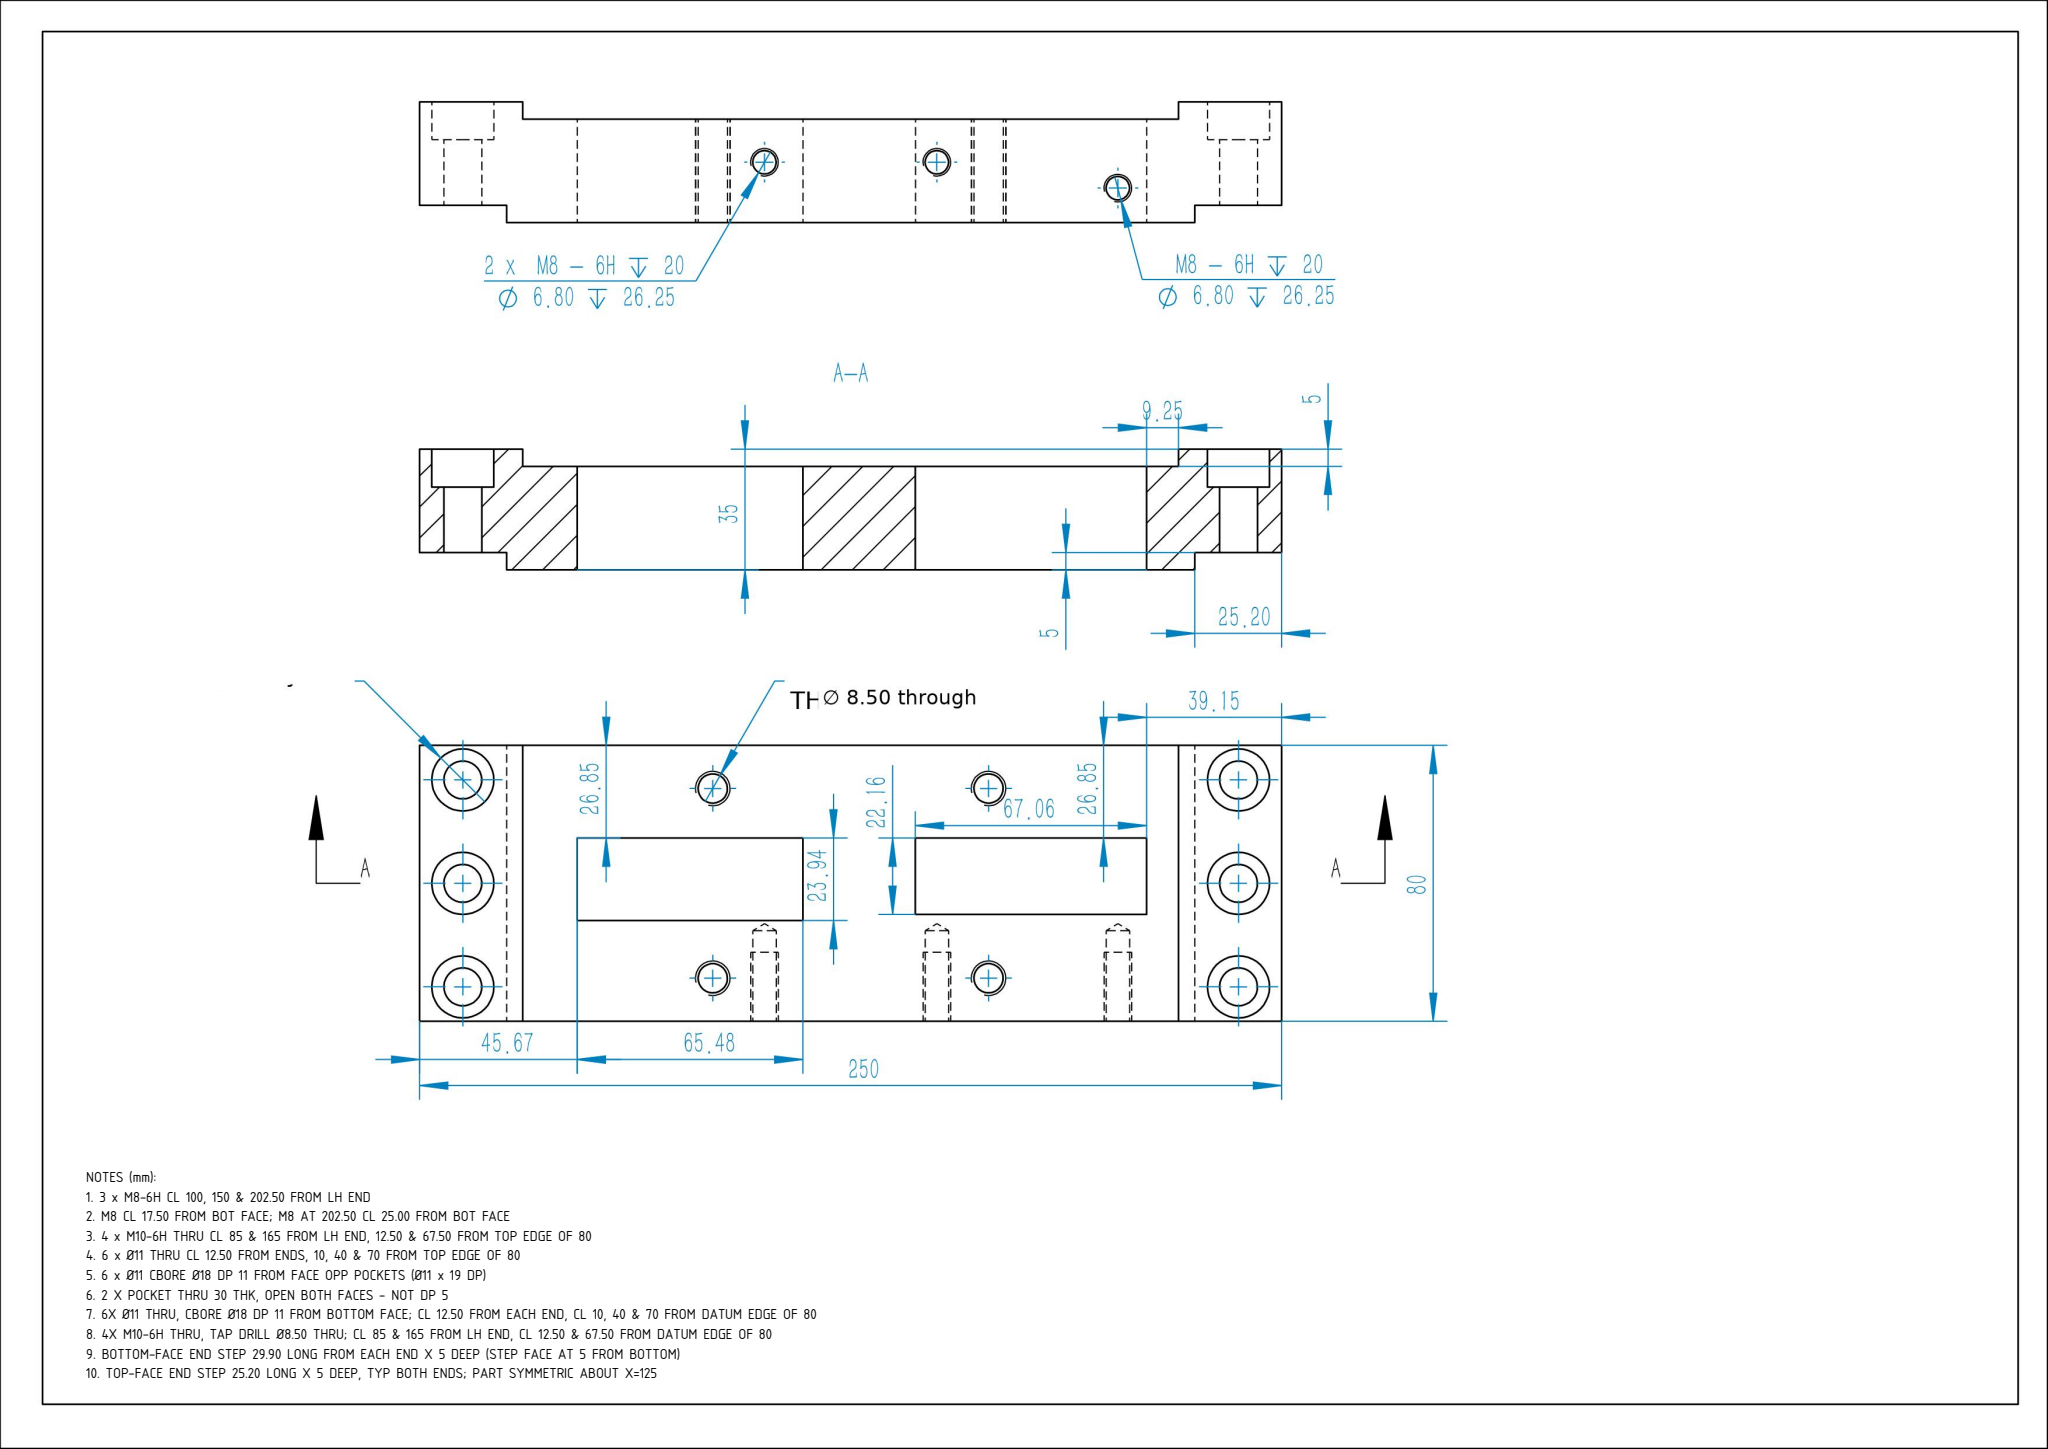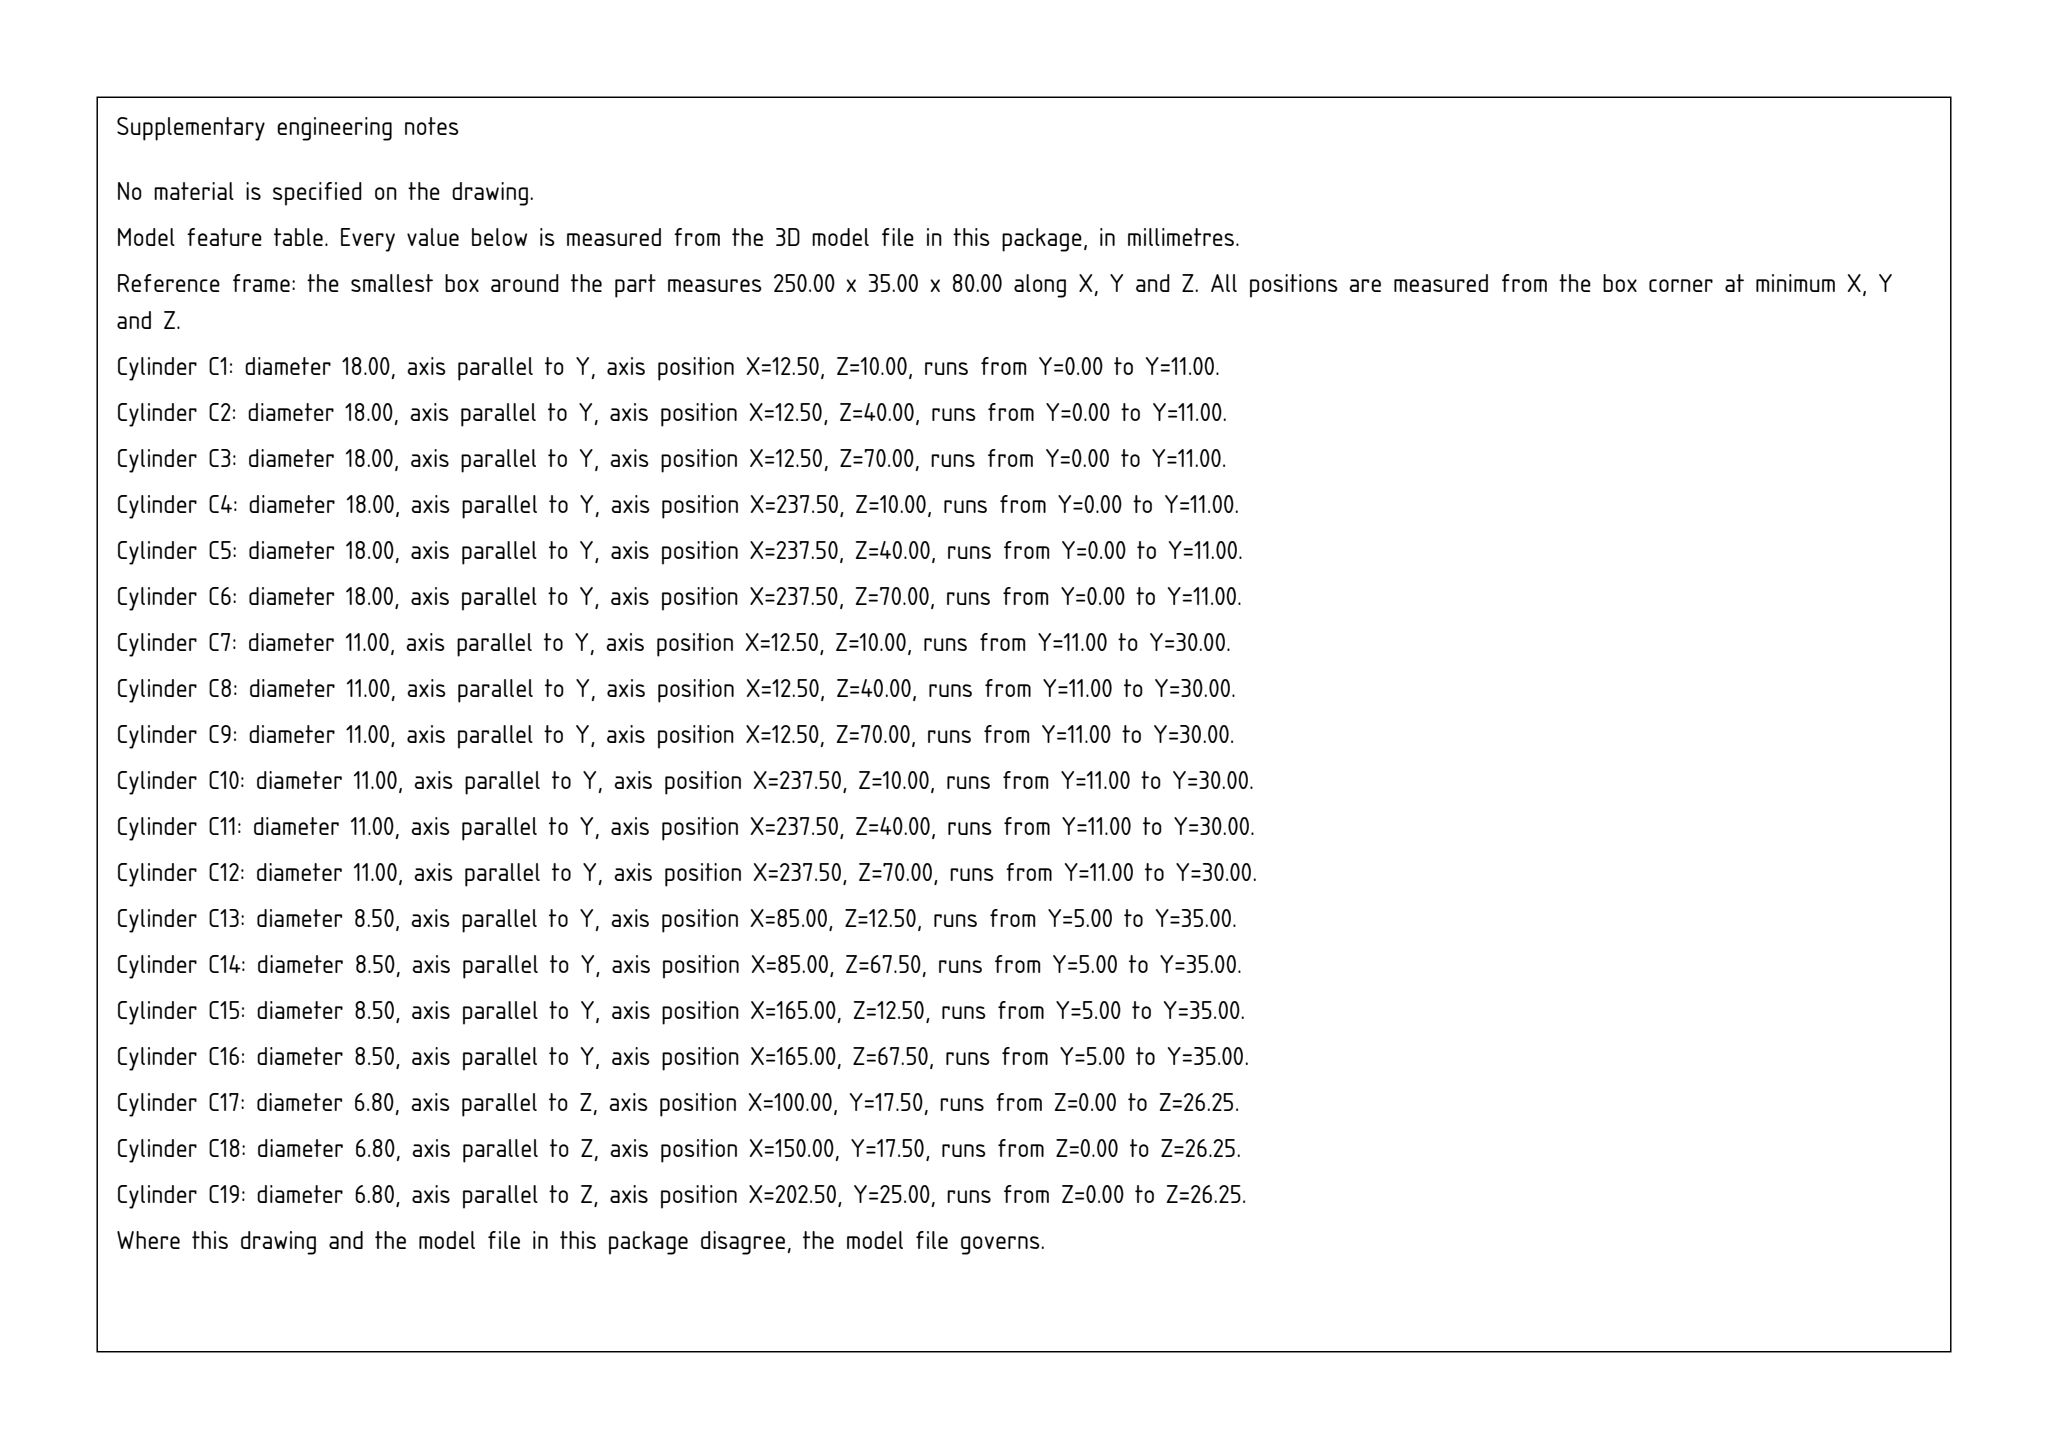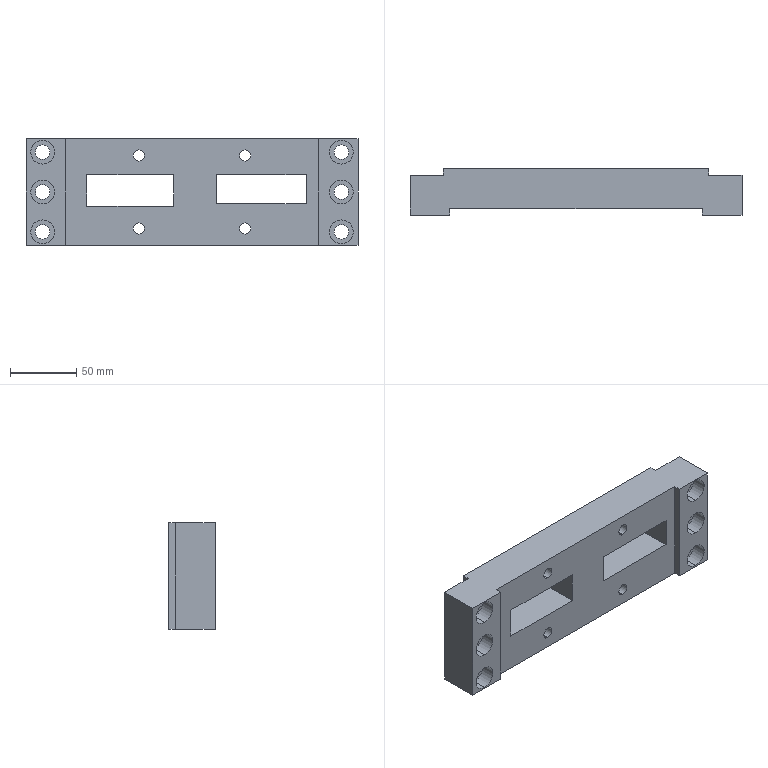Part | SolidWorks | mm | 1 solid | 72 faces | box 250 x 35 x 80 mm | volume 474796 mm3 | cylinder 38 | plane 28 | cone 6 | commonest cylinder face diameters 18 x12 11 x12 8.5 x8 6.8 x6
Drawing notes:
3 x M8-6H CL 100, 150 & 202.50 FROM LH END | from the solid: Ø6.80 cyls axis z at x=100, 150, 202.5, len 26.25
M8 CL 17.50 FROM BOT FACE; M8 AT 202.50 CL 25.00 FROM BOT FACE | from the solid: Ø6.80 axis z at y=17.5 (x100,150) and y=25.0 (x202.5)
4 x M10-6H THRU CL 85 & 165 FROM LH END, 12.50 & 67.50 FROM TOP EDGE OF 80 | from the solid: Ø8.5 axis y cyls at (85,12.5),(85,67.5),(165,12.5),(165,67.5), len 30
6 x Ø11 THRU CL 12.50 FROM ENDS, 10, 40 & 70 FROM TOP EDGE OF 80 | from the solid: Ø11 axis y cyls at x=12.5 & 237.5, z=10/40/70
6 x Ø11 CBORE Ø18 DP 11 FROM FACE OPP POCKETS (Ø11 x 19 DP) | from the solid: Ø18 cyl len 11 coaxial with Ø11 len 19; y-planes 0 & 11 (6 faces)
2 X POCKET THRU 30 THK, OPEN BOTH FACES - NOT DP 5 | from the solid: Pocket walls x45.7-111.2 & x143.8-210.9 span y 5.0 to 35.0 (full 30 web); floors only at z29.2/31.0 & 53.2, no y-floor face
6X Ø11 THRU, CBORE Ø18 DP 11 FROM BOTTOM FACE; CL 12.50 FROM EACH END, CL 10, 40 & 70 FROM DATUM EDGE OF 80 | from the solid: cylinders: Ø11 y-axis at x=12.5 & 237.5, z=10/40/70, y 11->30; Ø18 y-axis same x/z, y 0->11
4X M10-6H THRU, TAP DRILL Ø8.50 THRU; CL 85 & 165 FROM LH END, CL 12.50 & 67.50 FROM DATUM EDGE OF 80 | from the solid: cylinders: Ø8.5 y-axis at x=85 & 165, z=12.5 & 67.5, y 5->35
BOTTOM-FACE END STEP 29.90 LONG FROM EACH END X 5 DEEP (STEP FACE AT 5 FROM BOTTOM) | from the solid: axis_planes: y=0 faces x[0,29.9] & x[220.1,250]; y=5 face x[29.9,220.1]; x=29.9 and x=220.1 faces y[0,5]
TOP-FACE END STEP 25.20 LONG X 5 DEEP, TYP BOTH ENDS; PART SYMMETRIC ABOUT X=125 | from the solid: axis_planes: y=30 faces x[0,25.2] & x[224.8,250]; x=25.2 and x=224.8 faces y[30,35]
build123d program:
from build123d import *

# Parameters (mm, degrees)
SKETCH1_W                                          = 250
SKETCH1_H                                          = 80
BOSS_EXTRUDE1_DEPTH                                = 17.5
SKETCH6_W                                          = 190.2
SKETCH6_H                                          = 80
CUT_EXTRUDE1_DEPTH                                 = 5
SKETCH7_W                                          = 25.2
SKETCH7_H                                          = 80
CUT_EXTRUDE2_DEPTH                                 = 5
HOLE_SIZE_ACCORDING_TO_TYPE_1_OF_HEXAG_D           = 11
HOLE_SIZE_ACCORDING_TO_TYPE_1_OF_HEXAG_CBORE_D     = 18
HOLE_SIZE_ACCORDING_TO_TYPE_1_OF_HEXAG_CBORE_DEPTH = 11
M10_TAPPED_HOLE1_D                                 = 8.5
M8_TAPPED_HOLE1_D                                  = 6.8
M8_TAPPED_HOLE1_DEPTH                              = 26.25
M8_TAPPED_HOLE1_TIP                                = 2.043
M8_TAPPED_HOLE2_D                                  = 6.8
M8_TAPPED_HOLE2_DEPTH                              = 26.25
M8_TAPPED_HOLE2_TIP                                = 2.043
SKETCH16_W                                         = 65.478
SKETCH16_H                                         = 23.936
SKETCH16_W_2                                       = 67.061
SKETCH16_H_2                                       = 22.156
CUT_EXTRUDE3_DEPTH                                 = 94


with BuildPart() as part:
    # Sketch1 → Boss-Extrude1 (new, symmetric)
    with BuildSketch(Plane(origin=(0, 0, 0), x_dir=(1, 0, 0), z_dir=(0, 1, 0))):
        Rectangle(SKETCH1_W, SKETCH1_H)
    extrude(amount=BOSS_EXTRUDE1_DEPTH, both=True)

    # Sketch6 → Cut-Extrude1 (cut)
    with BuildSketch(Plane.XZ.offset(17.5)):
        Rectangle(SKETCH6_W, SKETCH6_H)
    extrude(amount=-CUT_EXTRUDE1_DEPTH, mode=Mode.SUBTRACT)

    # Sketch7 → Cut-Extrude2 (cut)
    with BuildSketch(Plane(origin=(0, 17.5, 0), x_dir=(1, 0, 0), z_dir=(0, 1, 0))):
        with Locations((-112.4, 0)):
            Rectangle(SKETCH7_W, SKETCH7_H)
        with Locations((112.4, 0)):
            Rectangle(SKETCH7_W, SKETCH7_H)
    extrude(amount=-CUT_EXTRUDE2_DEPTH, mode=Mode.SUBTRACT)

    # Hole Size _according to_ Type 1 of Hexag (through all)
    with Locations(Plane(origin=(0, -17.5, 0), x_dir=(-1, 0, 0), z_dir=(0, -1, 0))):
        with Locations((-112.5, 0), (-112.5, -30), (-112.5, 30), (112.5, 30), (112.5, -30), (112.5, 0)):
            CounterBoreHole(HOLE_SIZE_ACCORDING_TO_TYPE_1_OF_HEXAG_D / 2, HOLE_SIZE_ACCORDING_TO_TYPE_1_OF_HEXAG_CBORE_D / 2, HOLE_SIZE_ACCORDING_TO_TYPE_1_OF_HEXAG_CBORE_DEPTH)

    # M10 Tapped Hole1 (through all)
    with Locations(Plane(origin=(0, -12.5, 0), x_dir=(-1, 0, 0), z_dir=(0, -1, 0))):
        with Locations((40, -27.5), (-40, -27.5), (40, 27.5), (-40, 27.5)):
            Hole(M10_TAPPED_HOLE1_D / 2)

    # M8 Tapped Hole1
    with Locations(Plane(origin=(0, 0, -40), x_dir=(-1, 0, 0), z_dir=(0, 0, -1))):
        with Locations((25, 0), (-25, 0)):
            Hole(M8_TAPPED_HOLE1_D / 2, depth=M8_TAPPED_HOLE1_DEPTH)
            with Locations((0, 0, -(M8_TAPPED_HOLE1_DEPTH + M8_TAPPED_HOLE1_TIP / 2))):  # 118° drill point
                Cone(0, M8_TAPPED_HOLE1_D / 2, M8_TAPPED_HOLE1_TIP, mode=Mode.SUBTRACT)

    # M8 Tapped Hole2
    with Locations(Plane(origin=(0, 0, -40), x_dir=(-1, 0, 0), z_dir=(0, 0, -1))):
        with Locations((-77.5, 7.5)):
            Hole(M8_TAPPED_HOLE2_D / 2, depth=M8_TAPPED_HOLE2_DEPTH)
            with Locations((0, 0, -(M8_TAPPED_HOLE2_DEPTH + M8_TAPPED_HOLE2_TIP / 2))):  # 118° drill point
                Cone(0, M8_TAPPED_HOLE2_D / 2, M8_TAPPED_HOLE2_TIP, mode=Mode.SUBTRACT)

    # Sketch16 → Cut-Extrude3 (cut)
    with BuildSketch(Plane.XZ.offset(12.5)):
        with Locations((-46.586, 1.187)):
            Rectangle(SKETCH16_W, SKETCH16_H)
        with Locations((52.323, 2.077)):
            Rectangle(SKETCH16_W_2, SKETCH16_H_2)
    extrude(amount=-CUT_EXTRUDE3_DEPTH, mode=Mode.SUBTRACT)


solid = part.part